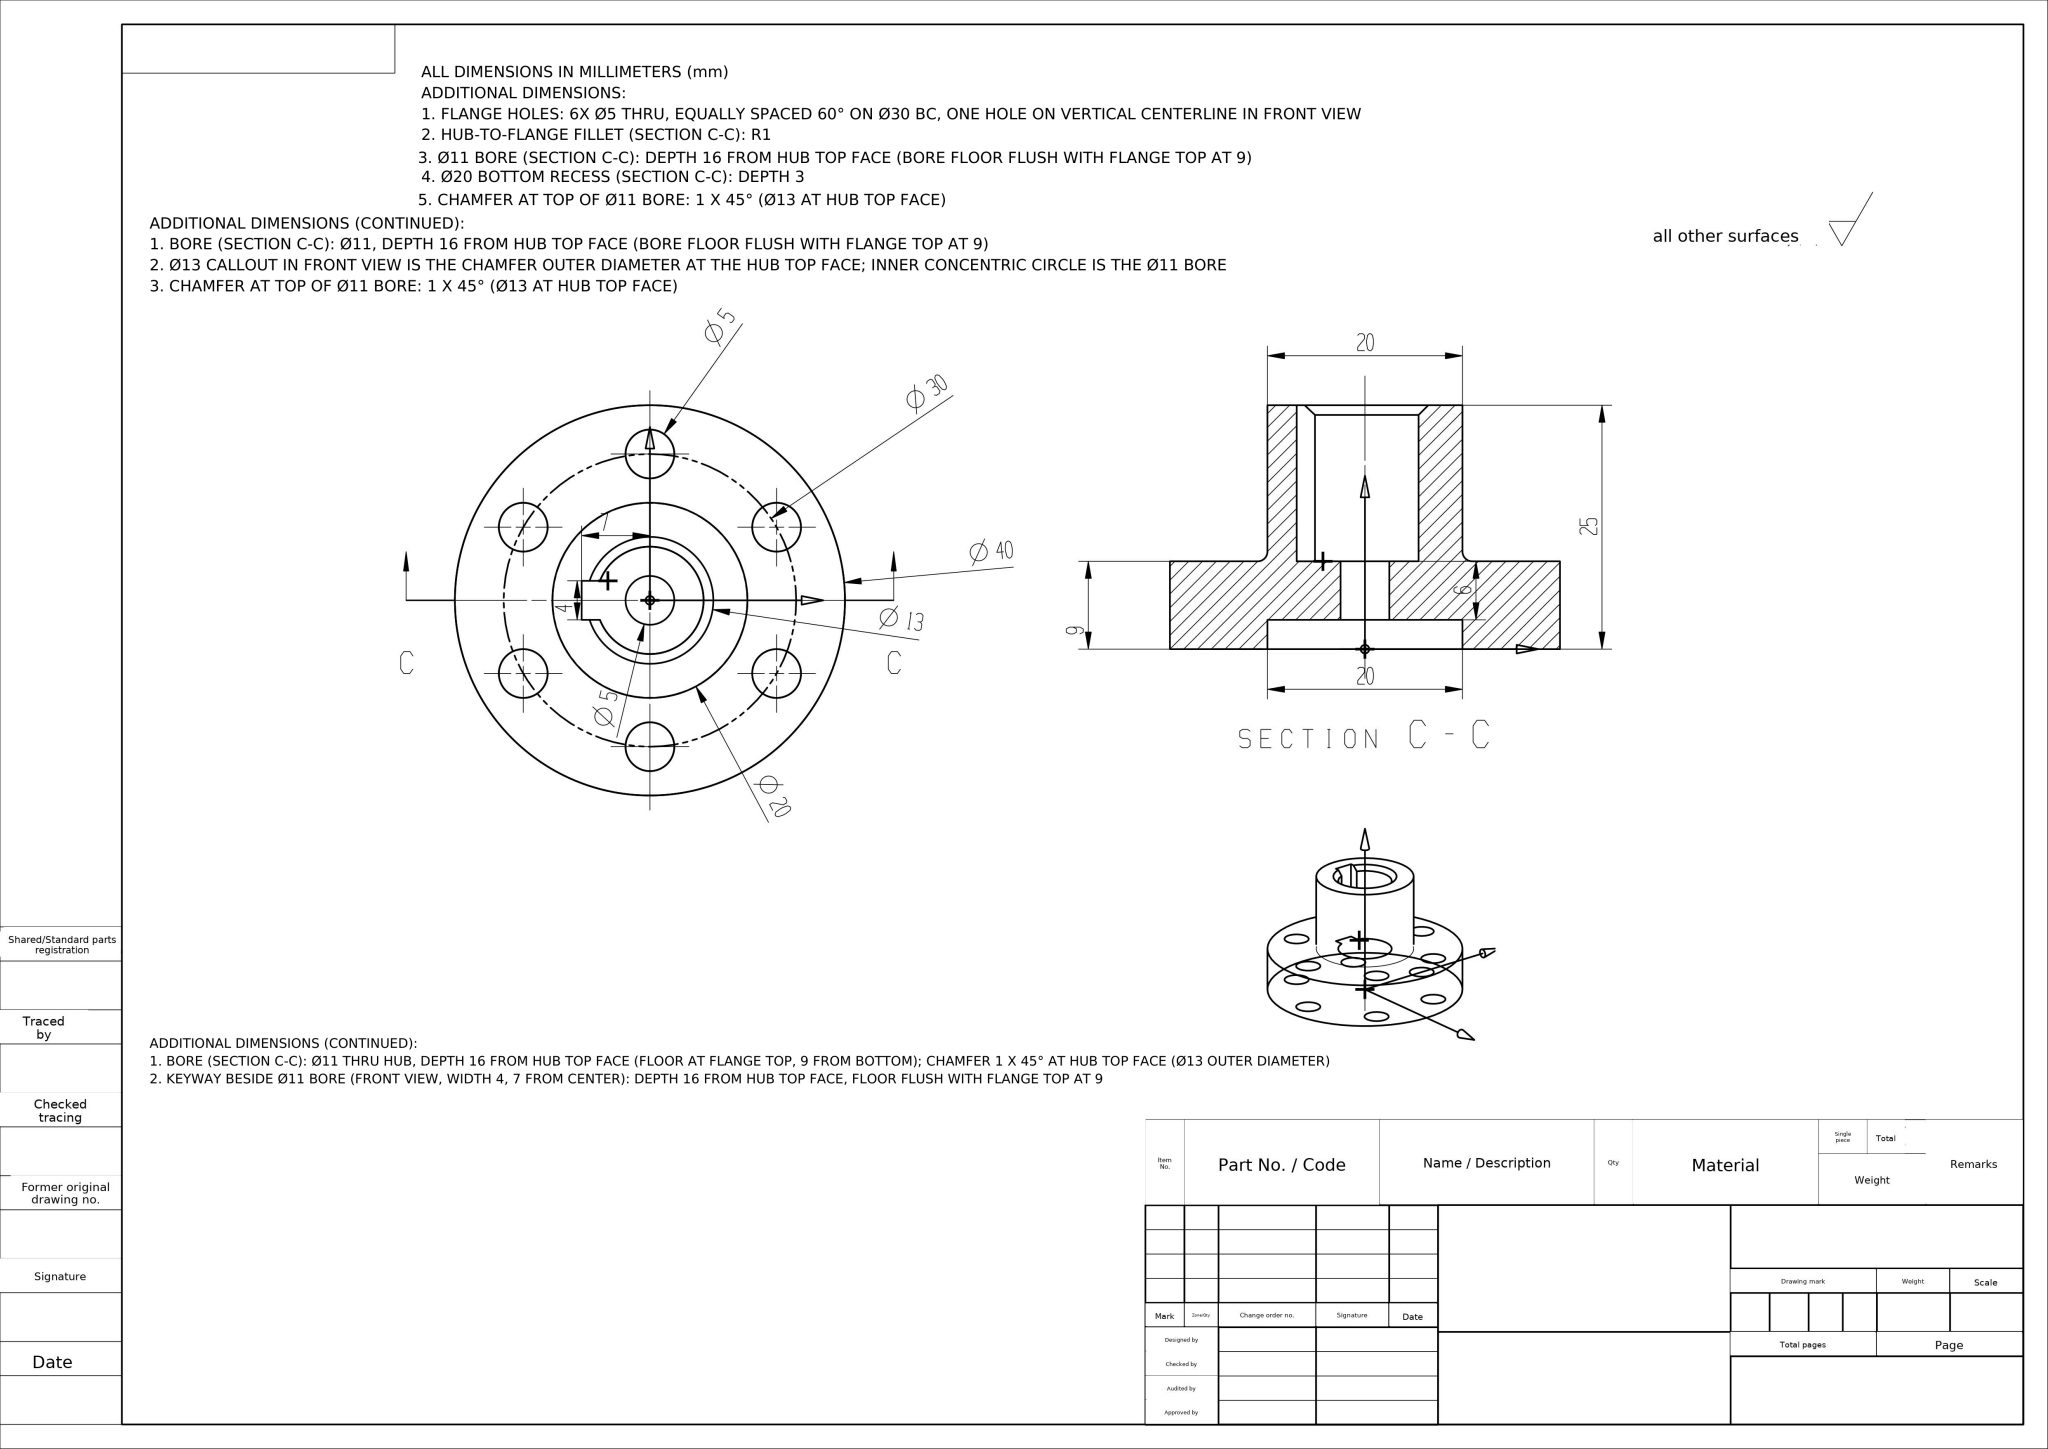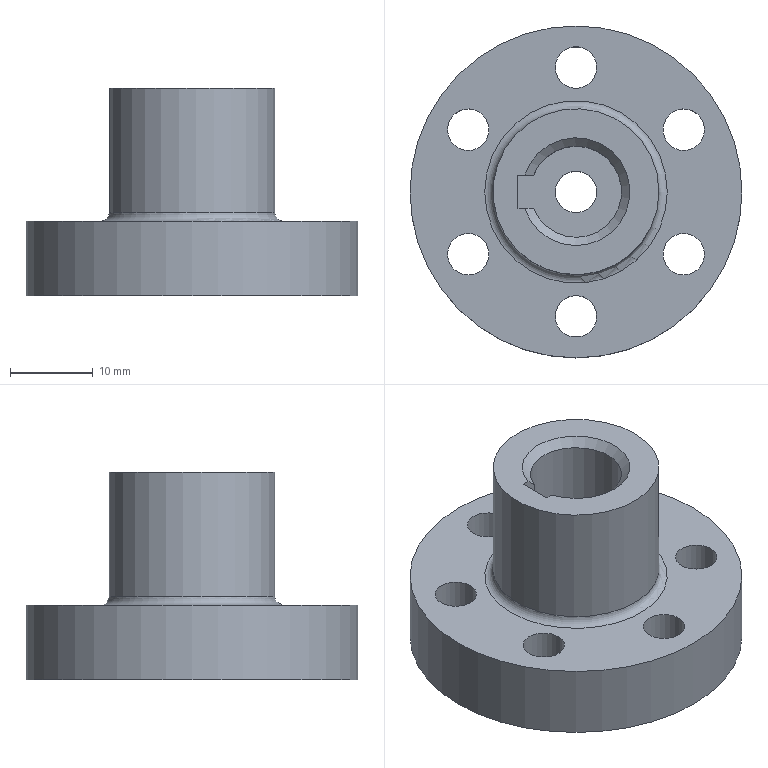Part | NX | mm | 1 solid | 21 faces | box 40 x 40 x 25 mm | volume 12589 mm3 | cylinder 11 | plane 8 | cone 1 | torus 1 | commonest cylinder face diameters 5 x7 20 x2 40 x1 11 x1
STEP:
#1=CARTESIAN_POINT('',(0.,0.,0.));
#2=DIRECTION('',(0.,0.,1.));
#3=DIRECTION('',(1.,0.,0.));
#4=AXIS2_PLACEMENT_3D('',#1,#2,#3);
#5=(LENGTH_UNIT()NAMED_UNIT(*)SI_UNIT(.MILLI.,.METRE.));
#6=UNCERTAINTY_MEASURE_WITH_UNIT(LENGTH_MEASURE(0.0508),#5,'','');
#7=(NAMED_UNIT(*)PLANE_ANGLE_UNIT()SI_UNIT($,.RADIAN.));
#8=PLANE_ANGLE_MEASURE_WITH_UNIT(PLANE_ANGLE_MEASURE(0.01745),#7);
#9=DIMENSIONAL_EXPONENTS(0.,0.,0.,0.,0.,0.,0.);
#10=(CONVERSION_BASED_UNIT('',#8)NAMED_UNIT(#9)PLANE_ANGLE_UNIT());
#11=(NAMED_UNIT(*)SI_UNIT($,.STERADIAN.)SOLID_ANGLE_UNIT());
#12=(GEOMETRIC_REPRESENTATION_CONTEXT(3)GLOBAL_UNCERTAINTY_ASSIGNED_CONTEXT((#6))GLOBAL_UNIT_ASSIGNED_CONTEXT((#5,#10,#11))REPRESENTATION_CONTEXT('',''));
#13=SHAPE_REPRESENTATION('',(#4),#12);
#14=CARTESIAN_POINT('',(10.,0.,25.));
#15=VERTEX_POINT('',#14);
#16=CARTESIAN_POINT('',(0.,0.,25.));
#17=DIRECTION('',(0.,0.,1.));
#18=DIRECTION('',(1.,0.,0.));
#19=AXIS2_PLACEMENT_3D('',#16,#17,#18);
#20=CIRCLE('',#19,10.);
#21=EDGE_CURVE('',#15,#15,#20,.T.);
#22=ORIENTED_EDGE('',*,*,#21,.T.);
#23=EDGE_LOOP('',(#22));
#24=FACE_BOUND('',#23,.T.);
#25=CARTESIAN_POINT('',(-7.,2.,25.));
#26=VERTEX_POINT('',#25);
#27=CARTESIAN_POINT('',(-6.185,2.,25.));
#28=VERTEX_POINT('',#27);
#29=CARTESIAN_POINT('',(-0.,2.,25.));
#30=DIRECTION('',(1.,0.,0.));
#31=VECTOR('',#30,1.);
#32=LINE('',#29,#31);
#33=EDGE_CURVE('',#26,#28,#32,.T.);
#34=ORIENTED_EDGE('',*,*,#33,.T.);
#35=CARTESIAN_POINT('',(-6.185,-2.,25.));
#36=VERTEX_POINT('',#35);
#37=CARTESIAN_POINT('',(0.,0.,25.));
#38=DIRECTION('',(0.,0.,-1.));
#39=DIRECTION('',(1.,0.,0.));
#40=AXIS2_PLACEMENT_3D('',#37,#38,#39);
#41=CIRCLE('',#40,6.5);
#42=EDGE_CURVE('',#28,#36,#41,.T.);
#43=ORIENTED_EDGE('',*,*,#42,.T.);
#44=CARTESIAN_POINT('',(-7.,-2.,25.));
#45=VERTEX_POINT('',#44);
#46=CARTESIAN_POINT('',(0.,-2.,25.));
#47=DIRECTION('',(-1.,0.,0.));
#48=VECTOR('',#47,1.);
#49=LINE('',#46,#48);
#50=EDGE_CURVE('',#36,#45,#49,.T.);
#51=ORIENTED_EDGE('',*,*,#50,.T.);
#52=CARTESIAN_POINT('',(-7.,-0.,25.));
#53=DIRECTION('',(-0.,1.,0.));
#54=VECTOR('',#53,1.);
#55=LINE('',#52,#54);
#56=EDGE_CURVE('',#45,#26,#55,.T.);
#57=ORIENTED_EDGE('',*,*,#56,.T.);
#58=EDGE_LOOP('',(#34,#43,#51,#57));
#59=FACE_BOUND('',#58,.T.);
#60=CARTESIAN_POINT('',(0.,0.,25.));
#61=DIRECTION('',(0.,0.,1.));
#62=DIRECTION('',(1.,0.,0.));
#63=AXIS2_PLACEMENT_3D('',#60,#61,#62);
#64=PLANE('',#63);
#65=ADVANCED_FACE('',(#24,#59),#64,.T.);
#66=CARTESIAN_POINT('',(-11.74,9.665,9.));
#67=VERTEX_POINT('',#66);
#68=CARTESIAN_POINT('',(-12.99,7.5,9.));
#69=DIRECTION('',(0.,0.,1.));
#70=DIRECTION('',(0.5,0.866,0.));
#71=AXIS2_PLACEMENT_3D('',#68,#69,#70);
#72=CIRCLE('',#71,2.5);
#73=EDGE_CURVE('',#67,#67,#72,.T.);
#74=ORIENTED_EDGE('',*,*,#73,.T.);
#75=EDGE_LOOP('',(#74));
#76=FACE_BOUND('',#75,.T.);
#77=CARTESIAN_POINT('',(-11.74,9.665,0.));
#78=VERTEX_POINT('',#77);
#79=CARTESIAN_POINT('',(-12.99,7.5,0.));
#80=DIRECTION('',(0.,0.,1.));
#81=DIRECTION('',(0.5,0.866,0.));
#82=AXIS2_PLACEMENT_3D('',#79,#80,#81);
#83=CIRCLE('',#82,2.5);
#84=EDGE_CURVE('',#78,#78,#83,.T.);
#85=ORIENTED_EDGE('',*,*,#84,.F.);
#86=EDGE_LOOP('',(#85));
#87=FACE_BOUND('',#86,.T.);
#88=CARTESIAN_POINT('',(-12.99,7.5,9.));
#89=DIRECTION('',(0.,0.,-1.));
#90=DIRECTION('',(-1.,0.,0.));
#91=AXIS2_PLACEMENT_3D('',#88,#89,#90);
#92=CYLINDRICAL_SURFACE('',#91,2.5);
#93=ADVANCED_FACE('',(#76,#87),#92,.F.);
#94=CARTESIAN_POINT('',(-2.5,-15.,9.));
#95=VERTEX_POINT('',#94);
#96=CARTESIAN_POINT('',(0.,-15.,9.));
#97=DIRECTION('',(0.,0.,1.));
#98=DIRECTION('',(-1.,0.,0.));
#99=AXIS2_PLACEMENT_3D('',#96,#97,#98);
#100=CIRCLE('',#99,2.5);
#101=EDGE_CURVE('',#95,#95,#100,.T.);
#102=ORIENTED_EDGE('',*,*,#101,.T.);
#103=EDGE_LOOP('',(#102));
#104=FACE_BOUND('',#103,.T.);
#105=CARTESIAN_POINT('',(-2.5,-15.,0.));
#106=VERTEX_POINT('',#105);
#107=CARTESIAN_POINT('',(0.,-15.,0.));
#108=DIRECTION('',(0.,0.,1.));
#109=DIRECTION('',(-1.,0.,0.));
#110=AXIS2_PLACEMENT_3D('',#107,#108,#109);
#111=CIRCLE('',#110,2.5);
#112=EDGE_CURVE('',#106,#106,#111,.T.);
#113=ORIENTED_EDGE('',*,*,#112,.F.);
#114=EDGE_LOOP('',(#113));
#115=FACE_BOUND('',#114,.T.);
#116=CARTESIAN_POINT('',(0.,-15.,9.));
#117=DIRECTION('',(0.,0.,-1.));
#118=DIRECTION('',(-1.,0.,0.));
#119=AXIS2_PLACEMENT_3D('',#116,#117,#118);
#120=CYLINDRICAL_SURFACE('',#119,2.5);
#121=ADVANCED_FACE('',(#104,#115),#120,.F.);
#122=CARTESIAN_POINT('',(2.5,15.,9.));
#123=VERTEX_POINT('',#122);
#124=CARTESIAN_POINT('',(0.,15.,9.));
#125=DIRECTION('',(0.,0.,1.));
#126=DIRECTION('',(1.,0.,0.));
#127=AXIS2_PLACEMENT_3D('',#124,#125,#126);
#128=CIRCLE('',#127,2.5);
#129=EDGE_CURVE('',#123,#123,#128,.T.);
#130=ORIENTED_EDGE('',*,*,#129,.T.);
#131=EDGE_LOOP('',(#130));
#132=FACE_BOUND('',#131,.T.);
#133=CARTESIAN_POINT('',(2.5,15.,0.));
#134=VERTEX_POINT('',#133);
#135=CARTESIAN_POINT('',(0.,15.,0.));
#136=DIRECTION('',(0.,0.,1.));
#137=DIRECTION('',(1.,0.,0.));
#138=AXIS2_PLACEMENT_3D('',#135,#136,#137);
#139=CIRCLE('',#138,2.5);
#140=EDGE_CURVE('',#134,#134,#139,.T.);
#141=ORIENTED_EDGE('',*,*,#140,.F.);
#142=EDGE_LOOP('',(#141));
#143=FACE_BOUND('',#142,.T.);
#144=CARTESIAN_POINT('',(0.,15.,9.));
#145=DIRECTION('',(0.,0.,-1.));
#146=DIRECTION('',(-1.,0.,0.));
#147=AXIS2_PLACEMENT_3D('',#144,#145,#146);
#148=CYLINDRICAL_SURFACE('',#147,2.5);
#149=ADVANCED_FACE('',(#132,#143),#148,.F.);
#150=CARTESIAN_POINT('',(11.74,-9.665,9.));
#151=VERTEX_POINT('',#150);
#152=CARTESIAN_POINT('',(12.99,-7.5,9.));
#153=DIRECTION('',(0.,0.,1.));
#154=DIRECTION('',(-0.5,-0.866,0.));
#155=AXIS2_PLACEMENT_3D('',#152,#153,#154);
#156=CIRCLE('',#155,2.5);
#157=EDGE_CURVE('',#151,#151,#156,.T.);
#158=ORIENTED_EDGE('',*,*,#157,.T.);
#159=EDGE_LOOP('',(#158));
#160=FACE_BOUND('',#159,.T.);
#161=CARTESIAN_POINT('',(11.74,-9.665,0.));
#162=VERTEX_POINT('',#161);
#163=CARTESIAN_POINT('',(12.99,-7.5,0.));
#164=DIRECTION('',(0.,0.,1.));
#165=DIRECTION('',(-0.5,-0.866,0.));
#166=AXIS2_PLACEMENT_3D('',#163,#164,#165);
#167=CIRCLE('',#166,2.5);
#168=EDGE_CURVE('',#162,#162,#167,.T.);
#169=ORIENTED_EDGE('',*,*,#168,.F.);
#170=EDGE_LOOP('',(#169));
#171=FACE_BOUND('',#170,.T.);
#172=CARTESIAN_POINT('',(12.99,-7.5,9.));
#173=DIRECTION('',(0.,0.,-1.));
#174=DIRECTION('',(-1.,0.,0.));
#175=AXIS2_PLACEMENT_3D('',#172,#173,#174);
#176=CYLINDRICAL_SURFACE('',#175,2.5);
#177=ADVANCED_FACE('',(#160,#171),#176,.F.);
#178=CARTESIAN_POINT('',(14.24,5.335,9.));
#179=VERTEX_POINT('',#178);
#180=CARTESIAN_POINT('',(12.99,7.5,9.));
#181=DIRECTION('',(0.,0.,1.));
#182=DIRECTION('',(0.5,-0.866,0.));
#183=AXIS2_PLACEMENT_3D('',#180,#181,#182);
#184=CIRCLE('',#183,2.5);
#185=EDGE_CURVE('',#179,#179,#184,.T.);
#186=ORIENTED_EDGE('',*,*,#185,.T.);
#187=EDGE_LOOP('',(#186));
#188=FACE_BOUND('',#187,.T.);
#189=CARTESIAN_POINT('',(14.24,5.335,0.));
#190=VERTEX_POINT('',#189);
#191=CARTESIAN_POINT('',(12.99,7.5,0.));
#192=DIRECTION('',(0.,0.,1.));
#193=DIRECTION('',(0.5,-0.866,0.));
#194=AXIS2_PLACEMENT_3D('',#191,#192,#193);
#195=CIRCLE('',#194,2.5);
#196=EDGE_CURVE('',#190,#190,#195,.T.);
#197=ORIENTED_EDGE('',*,*,#196,.F.);
#198=EDGE_LOOP('',(#197));
#199=FACE_BOUND('',#198,.T.);
#200=CARTESIAN_POINT('',(12.99,7.5,9.));
#201=DIRECTION('',(0.,0.,-1.));
#202=DIRECTION('',(-1.,0.,0.));
#203=AXIS2_PLACEMENT_3D('',#200,#201,#202);
#204=CYLINDRICAL_SURFACE('',#203,2.5);
#205=ADVANCED_FACE('',(#188,#199),#204,.F.);
#206=CARTESIAN_POINT('',(20.,0.,9.));
#207=VERTEX_POINT('',#206);
#208=CARTESIAN_POINT('',(0.,0.,9.));
#209=DIRECTION('',(0.,0.,1.));
#210=DIRECTION('',(1.,0.,0.));
#211=AXIS2_PLACEMENT_3D('',#208,#209,#210);
#212=CIRCLE('',#211,20.);
#213=EDGE_CURVE('',#207,#207,#212,.T.);
#214=ORIENTED_EDGE('',*,*,#213,.F.);
#215=EDGE_LOOP('',(#214));
#216=FACE_BOUND('',#215,.T.);
#217=CARTESIAN_POINT('',(20.,0.,0.));
#218=VERTEX_POINT('',#217);
#219=CARTESIAN_POINT('',(0.,0.,0.));
#220=DIRECTION('',(0.,0.,1.));
#221=DIRECTION('',(1.,0.,0.));
#222=AXIS2_PLACEMENT_3D('',#219,#220,#221);
#223=CIRCLE('',#222,20.);
#224=EDGE_CURVE('',#218,#218,#223,.T.);
#225=ORIENTED_EDGE('',*,*,#224,.T.);
#226=EDGE_LOOP('',(#225));
#227=FACE_BOUND('',#226,.T.);
#228=CARTESIAN_POINT('',(0.,0.,9.));
#229=DIRECTION('',(0.,0.,-1.));
#230=DIRECTION('',(-1.,0.,0.));
#231=AXIS2_PLACEMENT_3D('',#228,#229,#230);
#232=CYLINDRICAL_SURFACE('',#231,20.);
#233=ADVANCED_FACE('',(#216,#227),#232,.T.);
#234=CARTESIAN_POINT('',(-14.24,-5.335,9.));
#235=VERTEX_POINT('',#234);
#236=CARTESIAN_POINT('',(-12.99,-7.5,9.));
#237=DIRECTION('',(0.,0.,1.));
#238=DIRECTION('',(-0.5,0.866,0.));
#239=AXIS2_PLACEMENT_3D('',#236,#237,#238);
#240=CIRCLE('',#239,2.5);
#241=EDGE_CURVE('',#235,#235,#240,.T.);
#242=ORIENTED_EDGE('',*,*,#241,.T.);
#243=EDGE_LOOP('',(#242));
#244=FACE_BOUND('',#243,.T.);
#245=CARTESIAN_POINT('',(-14.24,-5.335,0.));
#246=VERTEX_POINT('',#245);
#247=CARTESIAN_POINT('',(-12.99,-7.5,0.));
#248=DIRECTION('',(0.,0.,1.));
#249=DIRECTION('',(-0.5,0.866,0.));
#250=AXIS2_PLACEMENT_3D('',#247,#248,#249);
#251=CIRCLE('',#250,2.5);
#252=EDGE_CURVE('',#246,#246,#251,.T.);
#253=ORIENTED_EDGE('',*,*,#252,.F.);
#254=EDGE_LOOP('',(#253));
#255=FACE_BOUND('',#254,.T.);
#256=CARTESIAN_POINT('',(-12.99,-7.5,9.));
#257=DIRECTION('',(0.,0.,-1.));
#258=DIRECTION('',(-1.,0.,0.));
#259=AXIS2_PLACEMENT_3D('',#256,#257,#258);
#260=CYLINDRICAL_SURFACE('',#259,2.5);
#261=ADVANCED_FACE('',(#244,#255),#260,.F.);
#262=CARTESIAN_POINT('',(11.,0.,9.));
#263=VERTEX_POINT('',#262);
#264=CARTESIAN_POINT('',(0.,0.,9.));
#265=DIRECTION('',(0.,0.,-1.));
#266=DIRECTION('',(1.,0.,0.));
#267=AXIS2_PLACEMENT_3D('',#264,#265,#266);
#268=CIRCLE('',#267,11.);
#269=EDGE_CURVE('',#263,#263,#268,.T.);
#270=ORIENTED_EDGE('',*,*,#269,.T.);
#271=EDGE_LOOP('',(#270));
#272=FACE_BOUND('',#271,.T.);
#273=ORIENTED_EDGE('',*,*,#213,.T.);
#274=EDGE_LOOP('',(#273));
#275=FACE_BOUND('',#274,.T.);
#276=ORIENTED_EDGE('',*,*,#185,.F.);
#277=EDGE_LOOP('',(#276));
#278=FACE_BOUND('',#277,.T.);
#279=ORIENTED_EDGE('',*,*,#157,.F.);
#280=EDGE_LOOP('',(#279));
#281=FACE_BOUND('',#280,.T.);
#282=ORIENTED_EDGE('',*,*,#129,.F.);
#283=EDGE_LOOP('',(#282));
#284=FACE_BOUND('',#283,.T.);
#285=ORIENTED_EDGE('',*,*,#101,.F.);
#286=EDGE_LOOP('',(#285));
#287=FACE_BOUND('',#286,.T.);
#288=ORIENTED_EDGE('',*,*,#73,.F.);
#289=EDGE_LOOP('',(#288));
#290=FACE_BOUND('',#289,.T.);
#291=ORIENTED_EDGE('',*,*,#241,.F.);
#292=EDGE_LOOP('',(#291));
#293=FACE_BOUND('',#292,.T.);
#294=CARTESIAN_POINT('',(6.495,3.75,9.));
#295=DIRECTION('',(0.,0.,1.));
#296=DIRECTION('',(1.,0.,0.));
#297=AXIS2_PLACEMENT_3D('',#294,#295,#296);
#298=PLANE('',#297);
#299=ADVANCED_FACE('',(#272,#275,#278,#281,#284,#287,#290,#293),#298,.T.);
#300=CARTESIAN_POINT('',(10.,0.,0.));
#301=VERTEX_POINT('',#300);
#302=CARTESIAN_POINT('',(0.,0.,0.));
#303=DIRECTION('',(0.,0.,1.));
#304=DIRECTION('',(1.,0.,0.));
#305=AXIS2_PLACEMENT_3D('',#302,#303,#304);
#306=CIRCLE('',#305,10.);
#307=EDGE_CURVE('',#301,#301,#306,.T.);
#308=ORIENTED_EDGE('',*,*,#307,.T.);
#309=EDGE_LOOP('',(#308));
#310=FACE_BOUND('',#309,.T.);
#311=ORIENTED_EDGE('',*,*,#224,.F.);
#312=EDGE_LOOP('',(#311));
#313=FACE_BOUND('',#312,.T.);
#314=ORIENTED_EDGE('',*,*,#196,.T.);
#315=EDGE_LOOP('',(#314));
#316=FACE_BOUND('',#315,.T.);
#317=ORIENTED_EDGE('',*,*,#168,.T.);
#318=EDGE_LOOP('',(#317));
#319=FACE_BOUND('',#318,.T.);
#320=ORIENTED_EDGE('',*,*,#140,.T.);
#321=EDGE_LOOP('',(#320));
#322=FACE_BOUND('',#321,.T.);
#323=ORIENTED_EDGE('',*,*,#112,.T.);
#324=EDGE_LOOP('',(#323));
#325=FACE_BOUND('',#324,.T.);
#326=ORIENTED_EDGE('',*,*,#84,.T.);
#327=EDGE_LOOP('',(#326));
#328=FACE_BOUND('',#327,.T.);
#329=ORIENTED_EDGE('',*,*,#252,.T.);
#330=EDGE_LOOP('',(#329));
#331=FACE_BOUND('',#330,.T.);
#332=CARTESIAN_POINT('',(6.495,3.75,0.));
#333=DIRECTION('',(0.,0.,1.));
#334=DIRECTION('',(1.,0.,0.));
#335=AXIS2_PLACEMENT_3D('',#332,#333,#334);
#336=PLANE('',#335);
#337=ADVANCED_FACE('',(#310,#313,#316,#319,#322,#325,#328,#331),#336,.F.);
#338=CARTESIAN_POINT('',(2.5,0.,3.));
#339=VERTEX_POINT('',#338);
#340=CARTESIAN_POINT('',(0.,0.,3.));
#341=DIRECTION('',(0.,0.,1.));
#342=DIRECTION('',(1.,0.,0.));
#343=AXIS2_PLACEMENT_3D('',#340,#341,#342);
#344=CIRCLE('',#343,2.5);
#345=EDGE_CURVE('',#339,#339,#344,.T.);
#346=ORIENTED_EDGE('',*,*,#345,.T.);
#347=EDGE_LOOP('',(#346));
#348=FACE_BOUND('',#347,.T.);
#349=CARTESIAN_POINT('',(10.,0.,3.));
#350=VERTEX_POINT('',#349);
#351=CARTESIAN_POINT('',(0.,0.,3.));
#352=DIRECTION('',(0.,0.,1.));
#353=DIRECTION('',(1.,0.,0.));
#354=AXIS2_PLACEMENT_3D('',#351,#352,#353);
#355=CIRCLE('',#354,10.);
#356=EDGE_CURVE('',#350,#350,#355,.T.);
#357=ORIENTED_EDGE('',*,*,#356,.F.);
#358=EDGE_LOOP('',(#357));
#359=FACE_BOUND('',#358,.T.);
#360=CARTESIAN_POINT('',(0.,0.,3.));
#361=DIRECTION('',(0.,0.,1.));
#362=DIRECTION('',(1.,0.,0.));
#363=AXIS2_PLACEMENT_3D('',#360,#361,#362);
#364=PLANE('',#363);
#365=ADVANCED_FACE('',(#348,#359),#364,.F.);
#366=ORIENTED_EDGE('',*,*,#356,.T.);
#367=EDGE_LOOP('',(#366));
#368=FACE_BOUND('',#367,.T.);
#369=ORIENTED_EDGE('',*,*,#307,.F.);
#370=EDGE_LOOP('',(#369));
#371=FACE_BOUND('',#370,.T.);
#372=CARTESIAN_POINT('',(0.,0.,0.));
#373=DIRECTION('',(0.,0.,1.));
#374=DIRECTION('',(1.,0.,0.));
#375=AXIS2_PLACEMENT_3D('',#372,#373,#374);
#376=CYLINDRICAL_SURFACE('',#375,10.);
#377=ADVANCED_FACE('',(#368,#371),#376,.F.);
#378=CARTESIAN_POINT('',(2.5,0.,9.));
#379=VERTEX_POINT('',#378);
#380=CARTESIAN_POINT('',(0.,0.,9.));
#381=DIRECTION('',(0.,0.,1.));
#382=DIRECTION('',(1.,0.,0.));
#383=AXIS2_PLACEMENT_3D('',#380,#381,#382);
#384=CIRCLE('',#383,2.5);
#385=EDGE_CURVE('',#379,#379,#384,.T.);
#386=ORIENTED_EDGE('',*,*,#385,.T.);
#387=EDGE_LOOP('',(#386));
#388=FACE_BOUND('',#387,.T.);
#389=ORIENTED_EDGE('',*,*,#345,.F.);
#390=EDGE_LOOP('',(#389));
#391=FACE_BOUND('',#390,.T.);
#392=CARTESIAN_POINT('',(0.,0.,0.));
#393=DIRECTION('',(0.,0.,1.));
#394=DIRECTION('',(1.,0.,0.));
#395=AXIS2_PLACEMENT_3D('',#392,#393,#394);
#396=CYLINDRICAL_SURFACE('',#395,2.5);
#397=ADVANCED_FACE('',(#388,#391),#396,.F.);
#398=CARTESIAN_POINT('',(10.,0.,10.));
#399=VERTEX_POINT('',#398);
#400=CARTESIAN_POINT('',(0.,0.,10.));
#401=DIRECTION('',(0.,0.,1.));
#402=DIRECTION('',(1.,0.,0.));
#403=AXIS2_PLACEMENT_3D('',#400,#401,#402);
#404=CIRCLE('',#403,10.);
#405=EDGE_CURVE('',#399,#399,#404,.T.);
#406=ORIENTED_EDGE('',*,*,#405,.T.);
#407=EDGE_LOOP('',(#406));
#408=FACE_BOUND('',#407,.T.);
#409=ORIENTED_EDGE('',*,*,#21,.F.);
#410=EDGE_LOOP('',(#409));
#411=FACE_BOUND('',#410,.T.);
#412=CARTESIAN_POINT('',(0.,0.,25.));
#413=DIRECTION('',(0.,0.,-1.));
#414=DIRECTION('',(-1.,0.,0.));
#415=AXIS2_PLACEMENT_3D('',#412,#413,#414);
#416=CYLINDRICAL_SURFACE('',#415,10.);
#417=ADVANCED_FACE('',(#408,#411),#416,.T.);
#418=CARTESIAN_POINT('',(-7.,-2.,9.));
#419=VERTEX_POINT('',#418);
#420=CARTESIAN_POINT('',(-7.,-2.,30.));
#421=DIRECTION('',(0.,0.,1.));
#422=VECTOR('',#421,1.);
#423=LINE('',#420,#422);
#424=EDGE_CURVE('',#419,#45,#423,.T.);
#425=ORIENTED_EDGE('',*,*,#424,.F.);
#426=CARTESIAN_POINT('',(-7.,2.,9.));
#427=VERTEX_POINT('',#426);
#428=CARTESIAN_POINT('',(-7.,2.,9.));
#429=DIRECTION('',(-0.,1.,0.));
#430=VECTOR('',#429,1.);
#431=LINE('',#428,#430);
#432=EDGE_CURVE('',#419,#427,#431,.T.);
#433=ORIENTED_EDGE('',*,*,#432,.T.);
#434=CARTESIAN_POINT('',(-7.,2.,30.));
#435=DIRECTION('',(0.,0.,1.));
#436=VECTOR('',#435,1.);
#437=LINE('',#434,#436);
#438=EDGE_CURVE('',#427,#26,#437,.T.);
#439=ORIENTED_EDGE('',*,*,#438,.T.);
#440=ORIENTED_EDGE('',*,*,#56,.F.);
#441=EDGE_LOOP('',(#425,#433,#439,#440));
#442=FACE_OUTER_BOUND('',#441,.T.);
#443=CARTESIAN_POINT('',(-7.,2.,30.));
#444=DIRECTION('',(1.,0.,0.));
#445=DIRECTION('',(-0.,1.,0.));
#446=AXIS2_PLACEMENT_3D('',#443,#444,#445);
#447=PLANE('',#446);
#448=ADVANCED_FACE('',(#442),#447,.T.);
#449=ORIENTED_EDGE('',*,*,#50,.F.);
#450=CARTESIAN_POINT('',(-5.123,-2.,24.));
#451=VERTEX_POINT('',#450);
#452=CARTESIAN_POINT('',(-6.185,-2.,25.));
#453=CARTESIAN_POINT('',(-5.833,-2.,24.665));
#454=CARTESIAN_POINT('',(-5.479,-2.,24.331));
#455=CARTESIAN_POINT('',(-5.123,-2.,24.));
#456=B_SPLINE_CURVE_WITH_KNOTS('',3,(#452,#453,#454,#455),.UNSPECIFIED.,.F.,.F.,(4,4),(0.,1.),.UNSPECIFIED.);
#457=EDGE_CURVE('',#36,#451,#456,.T.);
#458=ORIENTED_EDGE('',*,*,#457,.T.);
#459=CARTESIAN_POINT('',(-5.123,-2.,9.));
#460=VERTEX_POINT('',#459);
#461=CARTESIAN_POINT('',(-5.123,-2.,30.));
#462=DIRECTION('',(0.,0.,1.));
#463=VECTOR('',#462,1.);
#464=LINE('',#461,#463);
#465=EDGE_CURVE('',#460,#451,#464,.T.);
#466=ORIENTED_EDGE('',*,*,#465,.F.);
#467=CARTESIAN_POINT('',(-7.,-2.,9.));
#468=DIRECTION('',(-1.,0.,0.));
#469=VECTOR('',#468,1.);
#470=LINE('',#467,#469);
#471=EDGE_CURVE('',#460,#419,#470,.T.);
#472=ORIENTED_EDGE('',*,*,#471,.T.);
#473=ORIENTED_EDGE('',*,*,#424,.T.);
#474=EDGE_LOOP('',(#449,#458,#466,#472,#473));
#475=FACE_OUTER_BOUND('',#474,.T.);
#476=CARTESIAN_POINT('',(-7.,-2.,30.));
#477=DIRECTION('',(0.,1.,0.));
#478=DIRECTION('',(0.,0.,1.));
#479=AXIS2_PLACEMENT_3D('',#476,#477,#478);
#480=PLANE('',#479);
#481=ADVANCED_FACE('',(#475),#480,.T.);
#482=ORIENTED_EDGE('',*,*,#465,.T.);
#483=CARTESIAN_POINT('',(-5.123,2.,24.));
#484=VERTEX_POINT('',#483);
#485=CARTESIAN_POINT('',(0.,0.,24.));
#486=DIRECTION('',(0.,0.,1.));
#487=DIRECTION('',(1.,0.,0.));
#488=AXIS2_PLACEMENT_3D('',#485,#486,#487);
#489=CIRCLE('',#488,5.5);
#490=EDGE_CURVE('',#451,#484,#489,.T.);
#491=ORIENTED_EDGE('',*,*,#490,.T.);
#492=CARTESIAN_POINT('',(-5.123,2.,9.));
#493=VERTEX_POINT('',#492);
#494=CARTESIAN_POINT('',(-5.123,2.,30.));
#495=DIRECTION('',(0.,0.,1.));
#496=VECTOR('',#495,1.);
#497=LINE('',#494,#496);
#498=EDGE_CURVE('',#493,#484,#497,.T.);
#499=ORIENTED_EDGE('',*,*,#498,.F.);
#500=CARTESIAN_POINT('',(0.,0.,9.));
#501=DIRECTION('',(0.,0.,-1.));
#502=DIRECTION('',(1.,0.,0.));
#503=AXIS2_PLACEMENT_3D('',#500,#501,#502);
#504=CIRCLE('',#503,5.5);
#505=EDGE_CURVE('',#493,#460,#504,.T.);
#506=ORIENTED_EDGE('',*,*,#505,.T.);
#507=EDGE_LOOP('',(#482,#491,#499,#506));
#508=FACE_OUTER_BOUND('',#507,.T.);
#509=CARTESIAN_POINT('',(0.,0.,30.));
#510=DIRECTION('',(0.,0.,-1.));
#511=DIRECTION('',(-1.,0.,0.));
#512=AXIS2_PLACEMENT_3D('',#509,#510,#511);
#513=CYLINDRICAL_SURFACE('',#512,5.5);
#514=ADVANCED_FACE('',(#508),#513,.F.);
#515=ORIENTED_EDGE('',*,*,#498,.T.);
#516=CARTESIAN_POINT('',(-5.123,2.,24.));
#517=CARTESIAN_POINT('',(-5.479,2.,24.331));
#518=CARTESIAN_POINT('',(-5.833,2.,24.665));
#519=CARTESIAN_POINT('',(-6.185,2.,25.));
#520=B_SPLINE_CURVE_WITH_KNOTS('',3,(#516,#517,#518,#519),.UNSPECIFIED.,.F.,.F.,(4,4),(0.,1.),.UNSPECIFIED.);
#521=EDGE_CURVE('',#484,#28,#520,.T.);
#522=ORIENTED_EDGE('',*,*,#521,.T.);
#523=ORIENTED_EDGE('',*,*,#33,.F.);
#524=ORIENTED_EDGE('',*,*,#438,.F.);
#525=CARTESIAN_POINT('',(-5.123,2.,9.));
#526=DIRECTION('',(1.,0.,0.));
#527=VECTOR('',#526,1.);
#528=LINE('',#525,#527);
#529=EDGE_CURVE('',#427,#493,#528,.T.);
#530=ORIENTED_EDGE('',*,*,#529,.T.);
#531=EDGE_LOOP('',(#515,#522,#523,#524,#530));
#532=FACE_OUTER_BOUND('',#531,.T.);
#533=CARTESIAN_POINT('',(-5.123,2.,30.));
#534=DIRECTION('',(0.,-1.,0.));
#535=DIRECTION('',(1.,0.,0.));
#536=AXIS2_PLACEMENT_3D('',#533,#534,#535);
#537=PLANE('',#536);
#538=ADVANCED_FACE('',(#532),#537,.T.);
#539=ORIENTED_EDGE('',*,*,#385,.F.);
#540=EDGE_LOOP('',(#539));
#541=FACE_BOUND('',#540,.T.);
#542=ORIENTED_EDGE('',*,*,#432,.F.);
#543=ORIENTED_EDGE('',*,*,#471,.F.);
#544=ORIENTED_EDGE('',*,*,#505,.F.);
#545=ORIENTED_EDGE('',*,*,#529,.F.);
#546=EDGE_LOOP('',(#542,#543,#544,#545));
#547=FACE_BOUND('',#546,.T.);
#548=CARTESIAN_POINT('',(0.,0.,9.));
#549=DIRECTION('',(0.,0.,1.));
#550=DIRECTION('',(1.,0.,0.));
#551=AXIS2_PLACEMENT_3D('',#548,#549,#550);
#552=PLANE('',#551);
#553=ADVANCED_FACE('',(#541,#547),#552,.T.);
#554=ORIENTED_EDGE('',*,*,#521,.F.);
#555=ORIENTED_EDGE('',*,*,#490,.F.);
#556=ORIENTED_EDGE('',*,*,#457,.F.);
#557=ORIENTED_EDGE('',*,*,#42,.F.);
#558=EDGE_LOOP('',(#554,#555,#556,#557));
#559=FACE_OUTER_BOUND('',#558,.T.);
#560=CARTESIAN_POINT('',(0.,0.,25.));
#561=DIRECTION('',(0.,0.,1.));
#562=DIRECTION('',(1.,0.,-0.));
#563=AXIS2_PLACEMENT_3D('',#560,#561,#562);
#564=CONICAL_SURFACE('',#563,6.5,45.);
#565=ADVANCED_FACE('',(#559),#564,.F.);
#566=ORIENTED_EDGE('',*,*,#269,.F.);
#567=EDGE_LOOP('',(#566));
#568=FACE_BOUND('',#567,.T.);
#569=ORIENTED_EDGE('',*,*,#405,.F.);
#570=EDGE_LOOP('',(#569));
#571=FACE_BOUND('',#570,.T.);
#572=CARTESIAN_POINT('',(0.,0.,10.));
#573=DIRECTION('',(0.,0.,1.));
#574=DIRECTION('',(1.,0.,0.));
#575=AXIS2_PLACEMENT_3D('',#572,#573,#574);
#576=TOROIDAL_SURFACE('',#575,11.,1.);
#577=ADVANCED_FACE('',(#568,#571),#576,.F.);
#578=CLOSED_SHELL('',(#65,#93,#121,#149,#177,#205,#233,#261,#299,#337,#365,#377,#397,#417,#448,#481,#514,#538,#553,#565,#577));
#579=MANIFOLD_SOLID_BREP('',#578);
#580=ADVANCED_BREP_SHAPE_REPRESENTATION('',(#579),#12);
#581=SHAPE_REPRESENTATION_RELATIONSHIP('','',#13,#580);
#582=PRESENTATION_LAYER_ASSIGNMENT('','',(#579));
#583=COLOUR_RGB('',1.,0.6,0.);
#584=FILL_AREA_STYLE_COLOUR('',#583);
#585=FILL_AREA_STYLE('',(#584));
#586=SURFACE_STYLE_FILL_AREA(#585);
#587=SURFACE_SIDE_STYLE('',(#586));
#588=SURFACE_STYLE_USAGE(.BOTH.,#587);
#589=PRESENTATION_STYLE_ASSIGNMENT((#588));
#590=STYLED_ITEM('',(#589),#579);
#591=MECHANICAL_DESIGN_GEOMETRIC_PRESENTATION_REPRESENTATION('',(#590),#12);